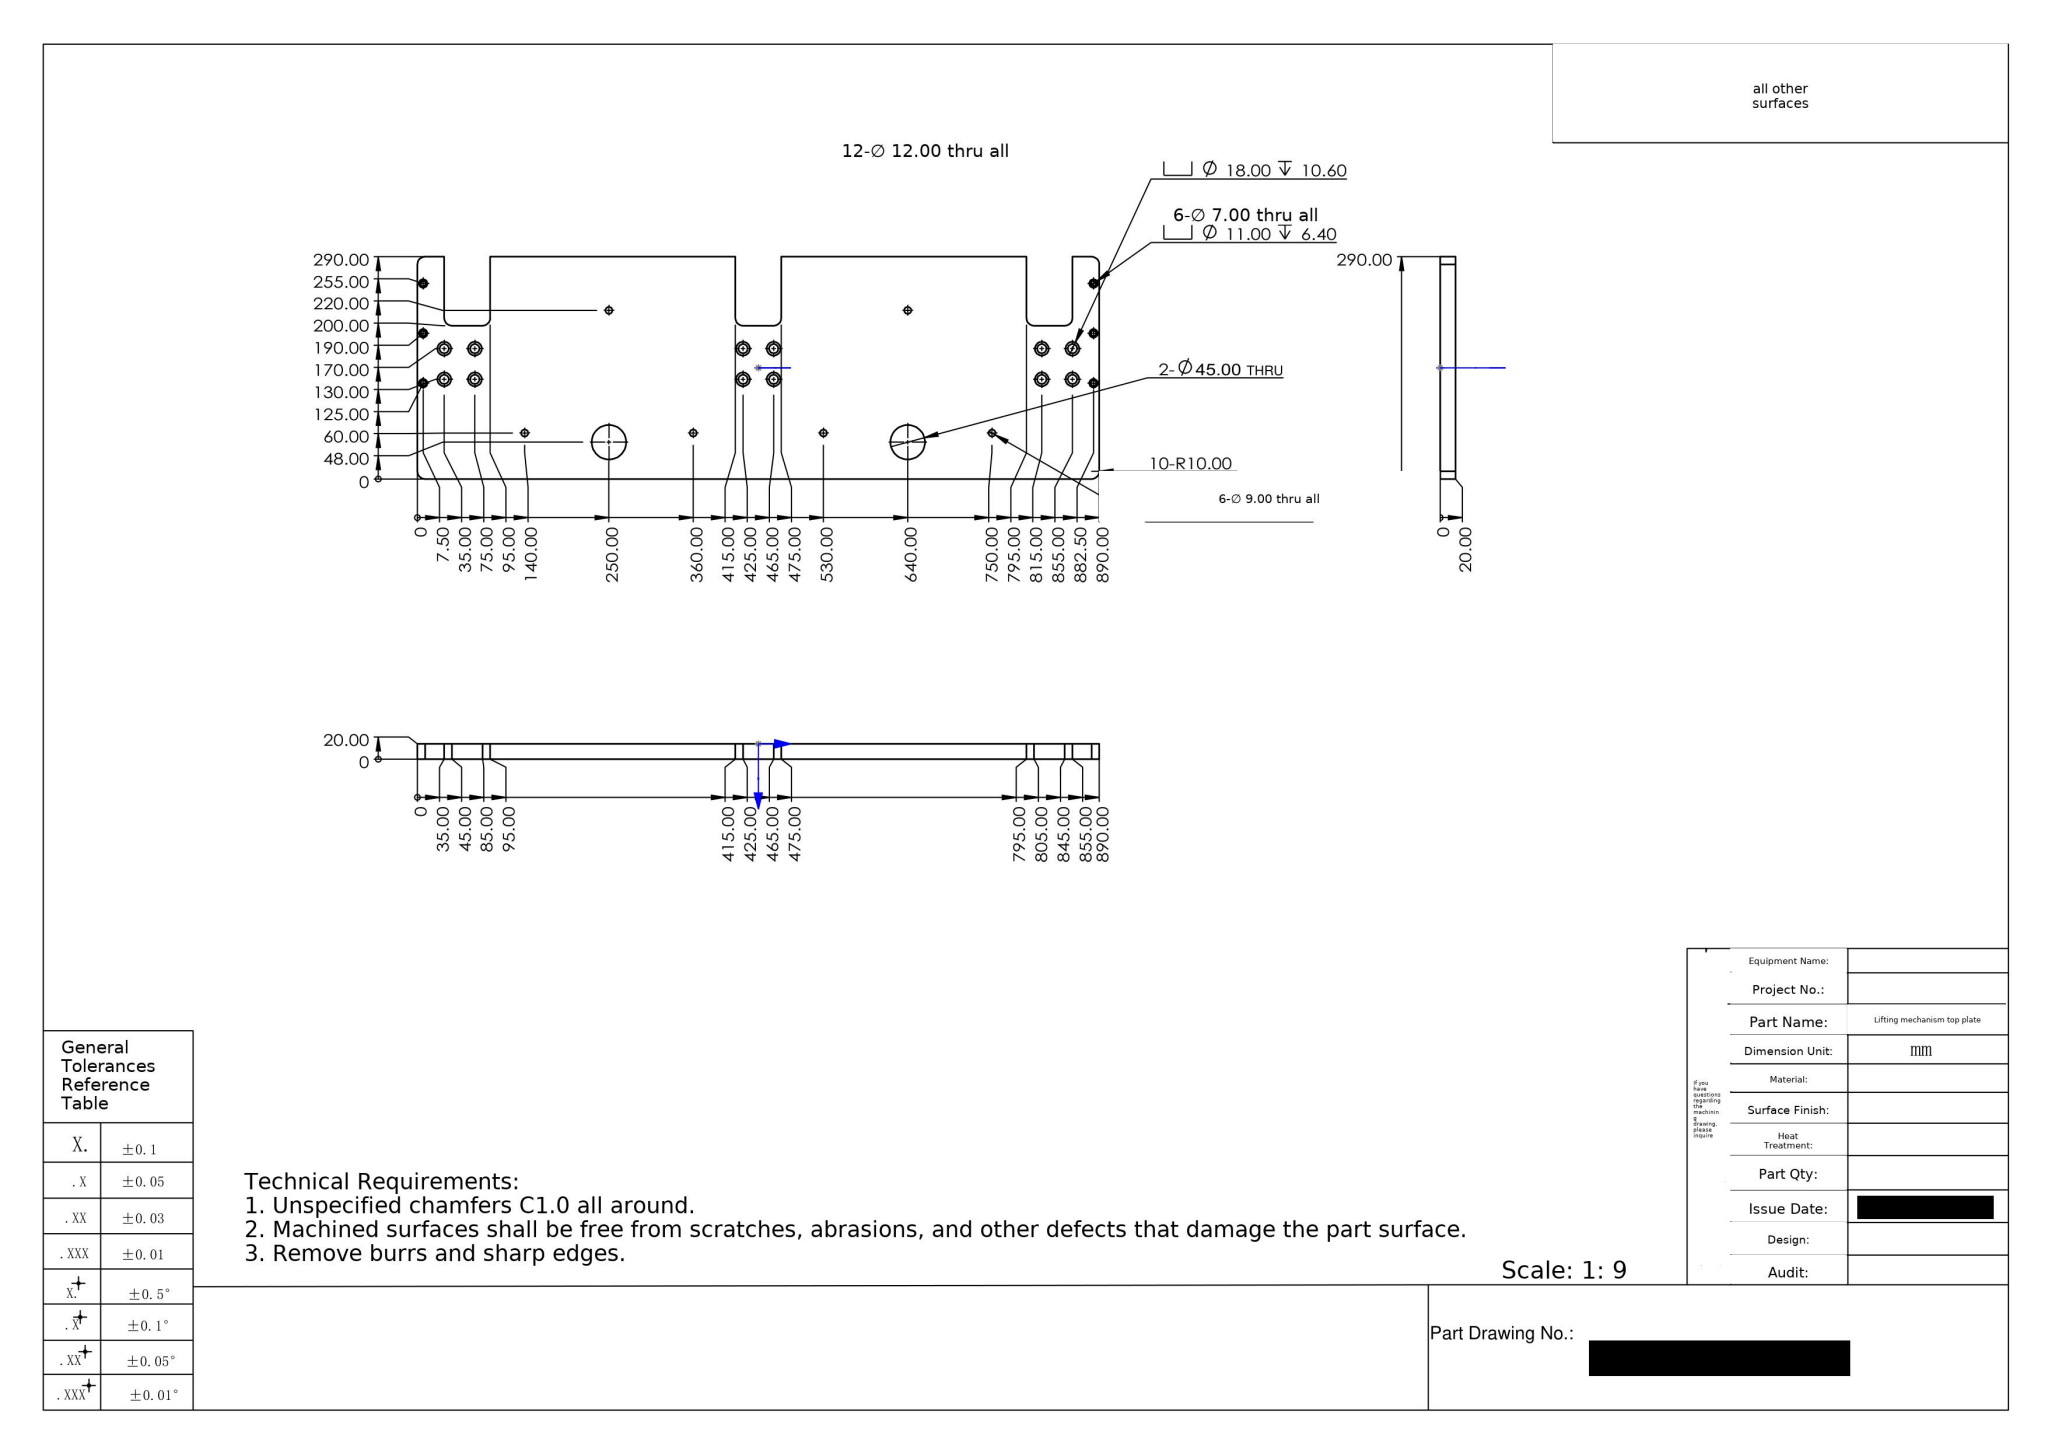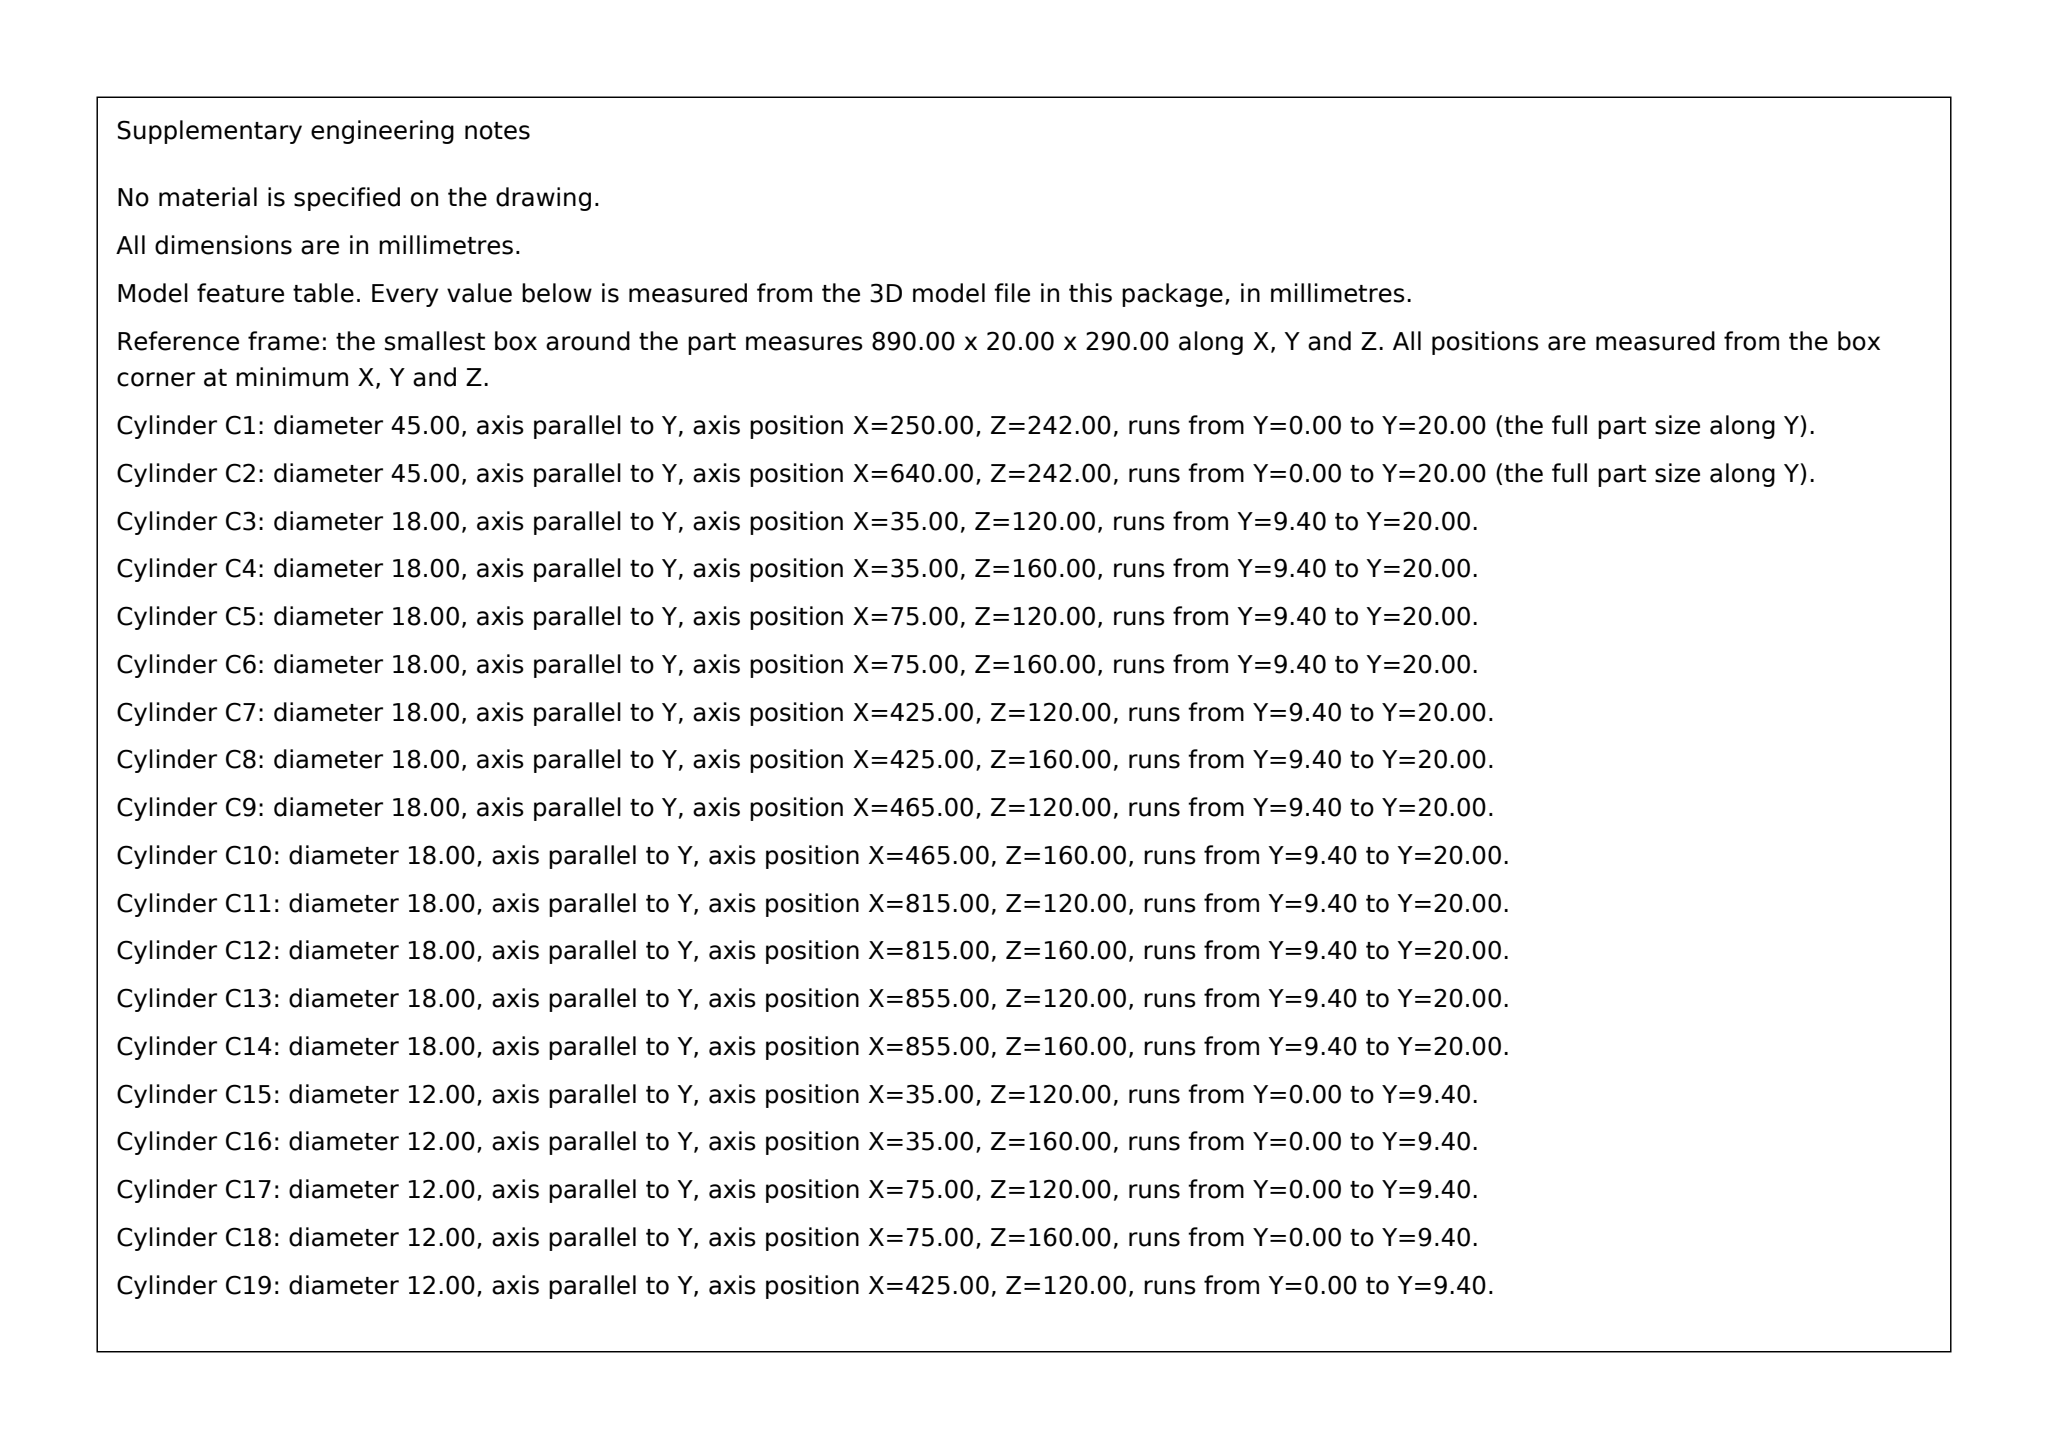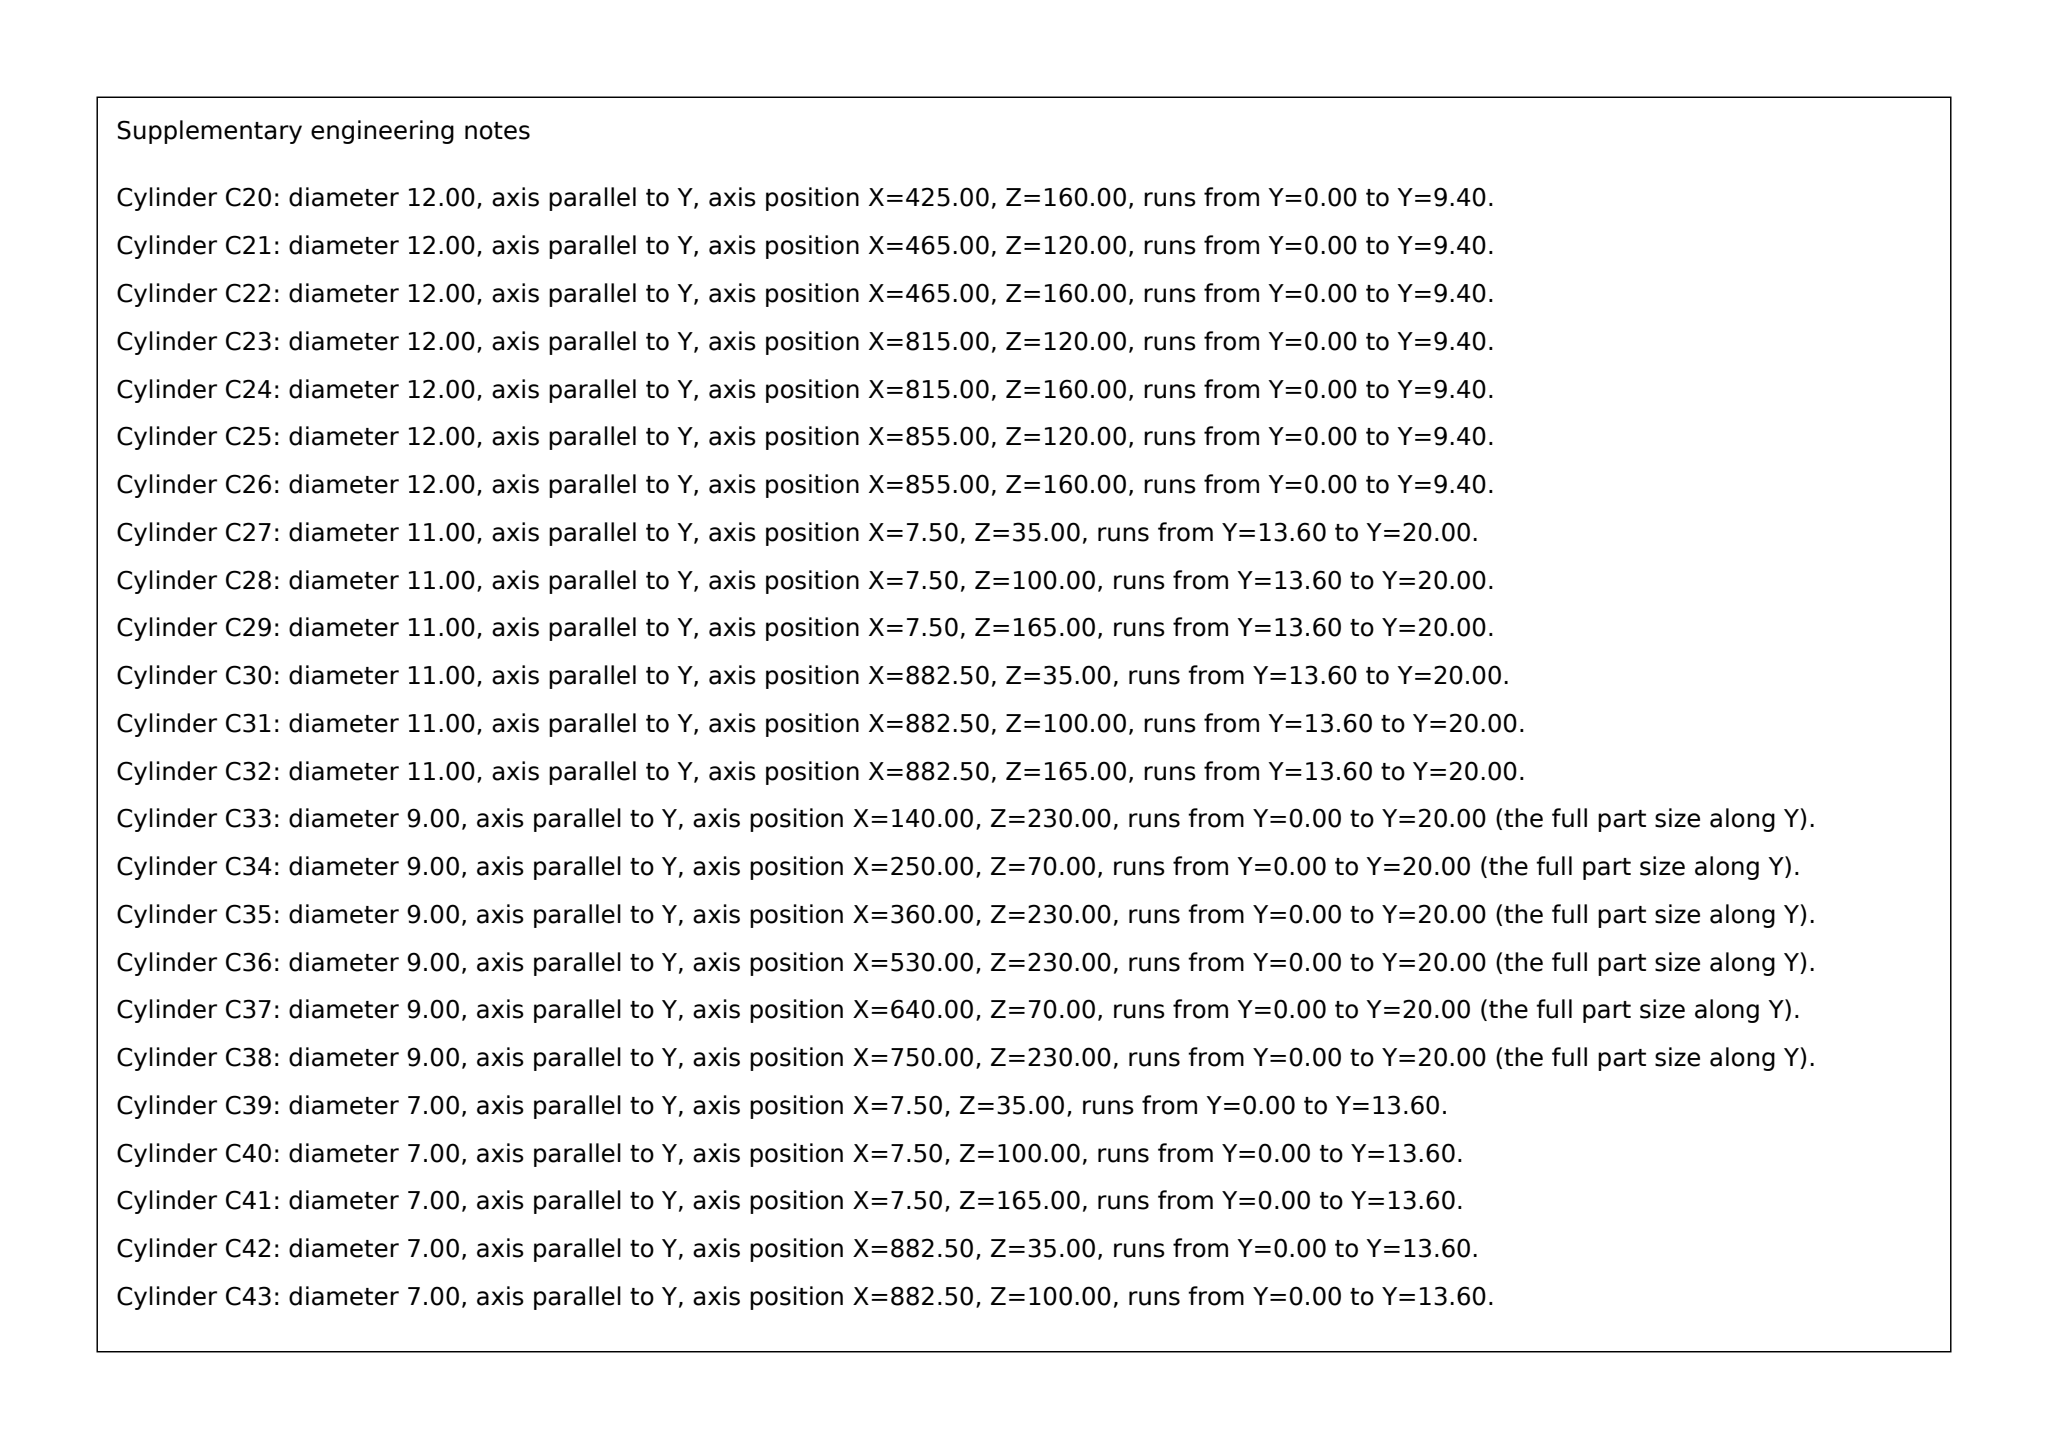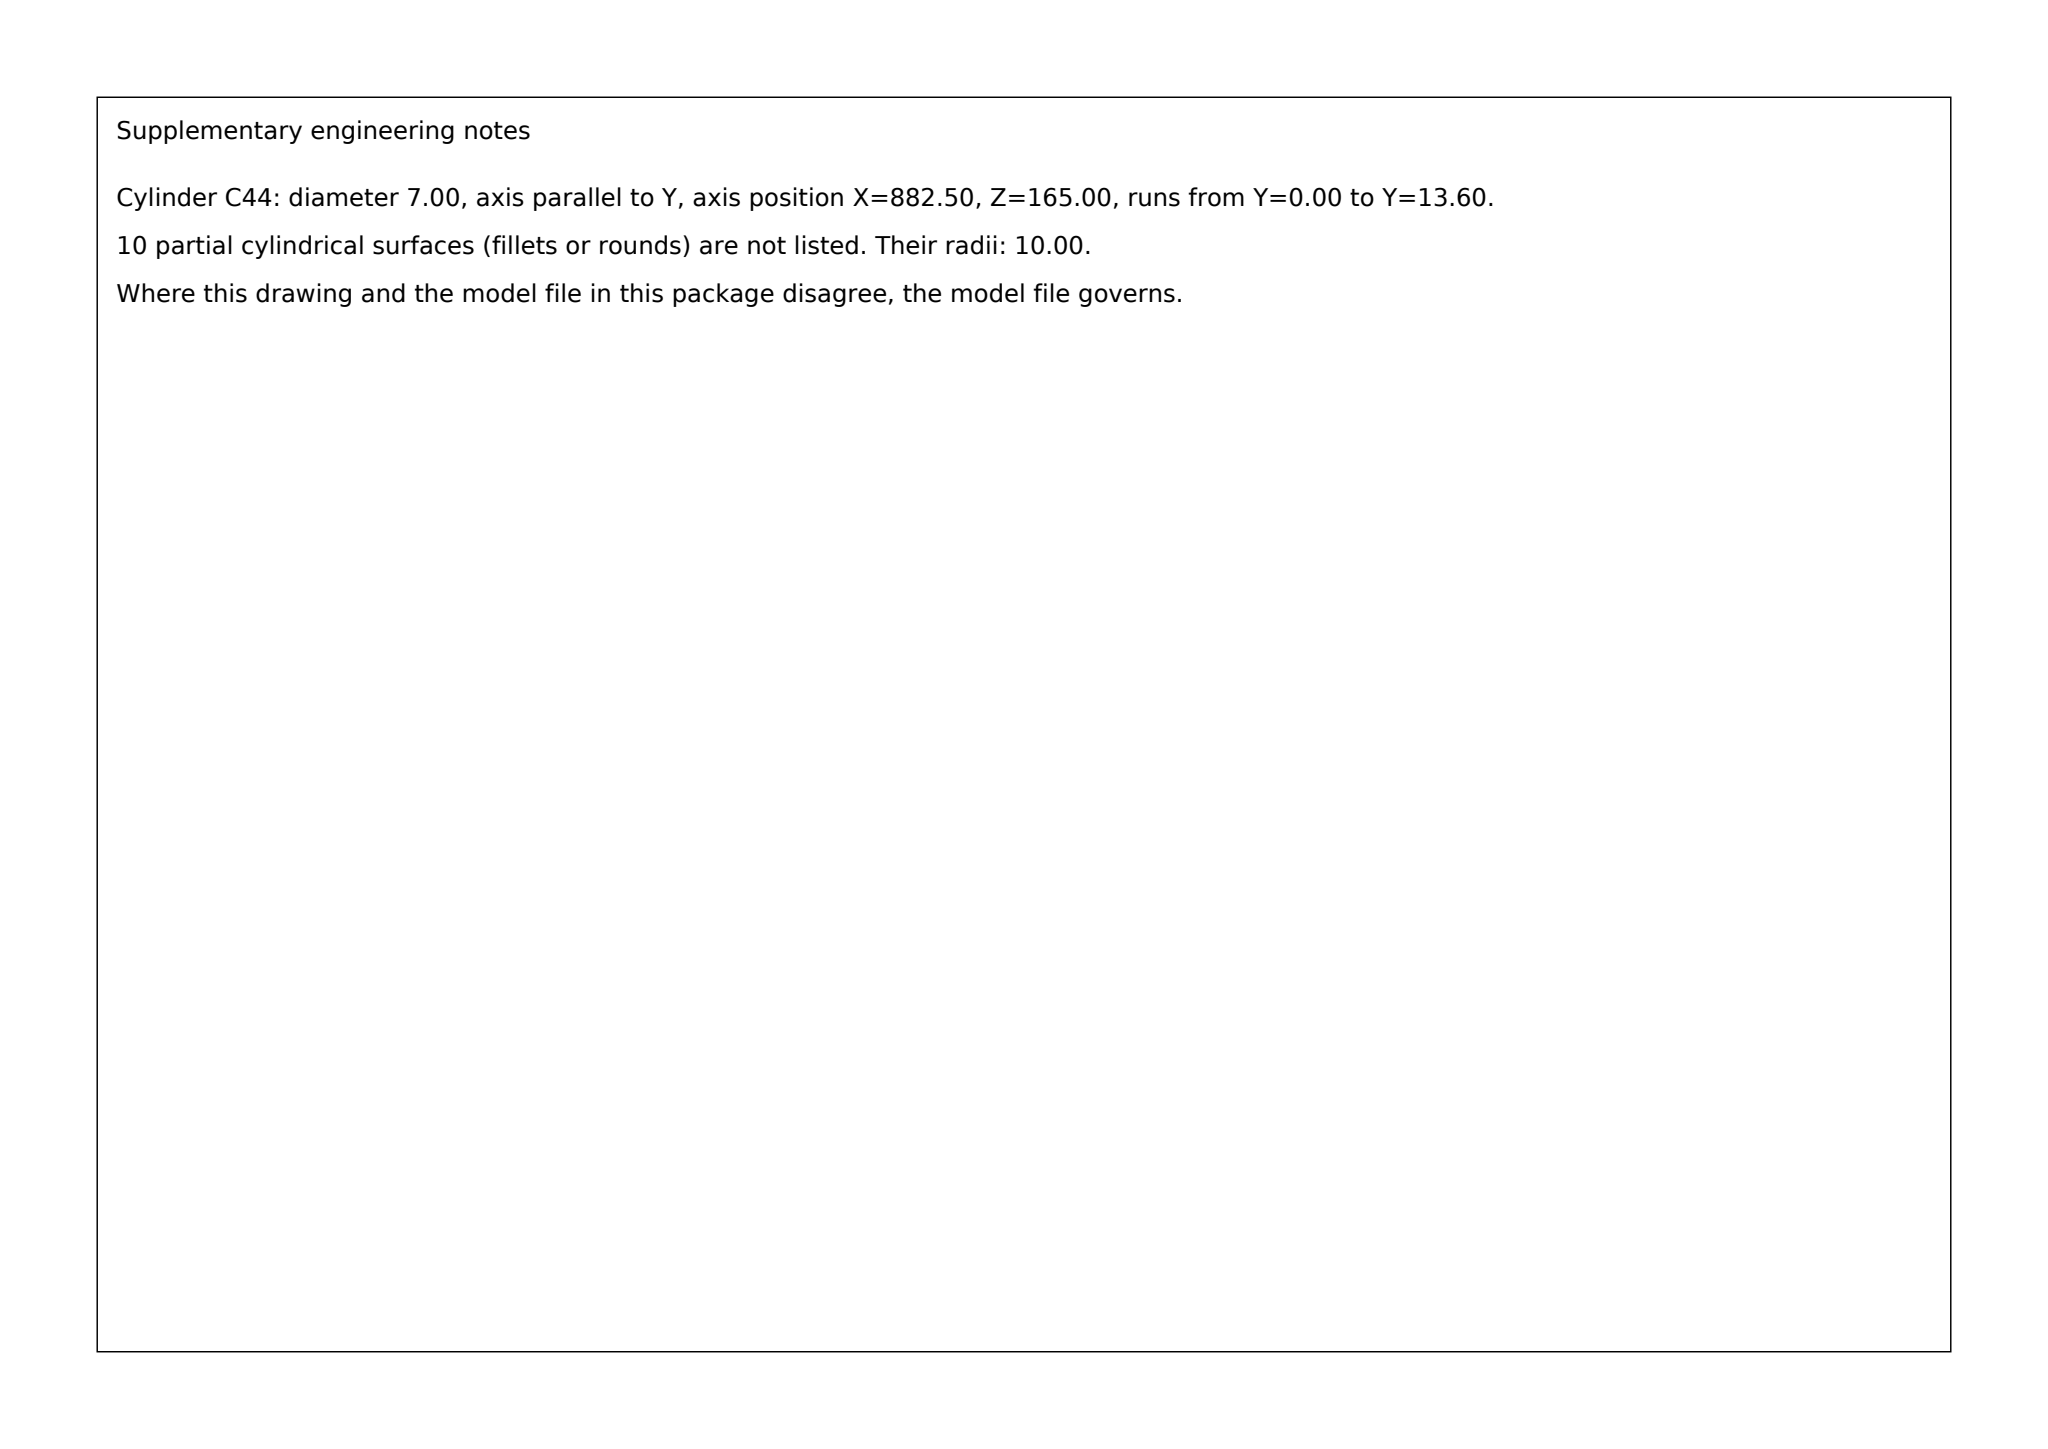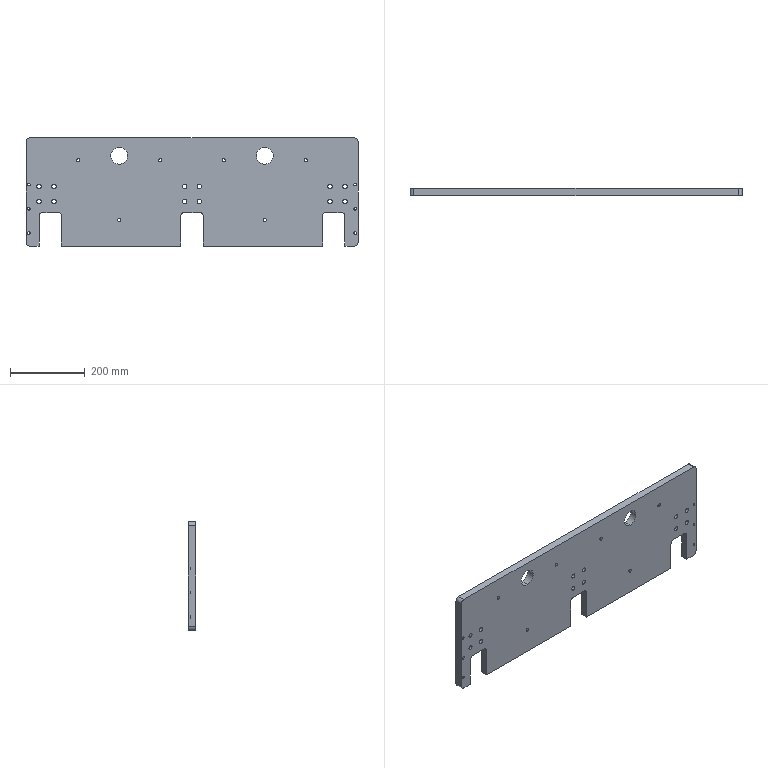Part | SolidWorks | mm | 1 solid | 134 faces | box 890 x 20 x 290 mm | volume 4715692 mm3 | cylinder 98 | plane 36 | commonest cylinder face diameters 18 x24 12 x24 11 x12 7 x12 9 x12 20 x10 45 x4
build123d program:
from build123d import *

# Parameters (mm, degrees)
SKETCH1_W                                        = 890
SKETCH1_H                                        = 290
BOSS_EXTRUDE1_DEPTH                              = 20
M8_CLEARANCE_HOLE2_D                             = 9
CUT_EXTRUDE1_DEPTH                               = 469.455
FILLET2_R                                        = 10
SKETCH15_R                                       = 22.5
CUT_EXTRUDE2_DEPTH                               = 469.455
M6_HEX_SOCKET_HEAD_CAP_SCREW_CBORE1_D            = 7
M6_HEX_SOCKET_HEAD_CAP_SCREW_CBORE1_CBORE_D      = 11
M6_HEX_SOCKET_HEAD_CAP_SCREW_CBORE1_CBORE_DEPTH  = 6.4
M10_HEX_SOCKET_HEAD_CAP_SCREW_CBORE1_D           = 12
M10_HEX_SOCKET_HEAD_CAP_SCREW_CBORE1_CBORE_D     = 18
M10_HEX_SOCKET_HEAD_CAP_SCREW_CBORE1_CBORE_DEPTH = 10.6


with BuildPart() as part:
    # Sketch1 → Boss-Extrude1 (new body)
    with BuildSketch(Plane(origin=(0, 0, 0), x_dir=(1, 0, 0), z_dir=(0, 1, 0))):
        Rectangle(SKETCH1_W, SKETCH1_H)
    extrude(amount=BOSS_EXTRUDE1_DEPTH)

    # M8 Clearance Hole2 (through all)
    with Locations(Plane(origin=(0, 20, 0), x_dir=(1, 0, 0), z_dir=(0, 1, 0))):
        with Locations((195, 75), (-195, 75), (-305, -85), (-85, -85), (85, -85), (305, -85)):
            Hole(M8_CLEARANCE_HOLE2_D / 2)

    # Sketch14 → Cut-Extrude1 (cut, through all)
    with BuildSketch(Plane(origin=(0, 20, 0), x_dir=(1, 0, 0), z_dir=(0, 1, 0))):
        with BuildLine():
            Line((-30, 145), (30, 145))
            Line((30, 145), (30, 65))
            ThreePointArc((30, 65), (27.071, 57.929), (20, 55))
            Line((20, 55), (-20, 55))
            ThreePointArc((-20, 55), (-27.071, 57.929), (-30, 65))
            Line((-30, 65), (-30, 145))
        make_face()
        with BuildLine():
            Line((-410, 145), (-350, 145))
            Line((-350, 145), (-350, 65))
            ThreePointArc((-350, 65), (-352.929, 57.929), (-360, 55))
            Line((-360, 55), (-400, 55))
            ThreePointArc((-400, 55), (-407.071, 57.929), (-410, 65))
            Line((-410, 65), (-410, 145))
        make_face()
        with BuildLine():
            Line((350, 145), (410, 145))
            Line((410, 145), (410, 65))
            ThreePointArc((410, 65), (407.071, 57.929), (400, 55))
            Line((400, 55), (360, 55))
            ThreePointArc((360, 55), (352.929, 57.929), (350, 65))
            Line((350, 65), (350, 145))
        make_face()
    extrude(amount=-CUT_EXTRUDE1_DEPTH, mode=Mode.SUBTRACT)

    # Fillet2
    fillet2_edges = [part.edges().sort_by_distance(p)[0] for p in [
        (-445, 10, -145),
        (445, 10, -145),
        (445, 10, 145),
        (-445, 10, 145),
    ]]
    fillet(fillet2_edges, radius=FILLET2_R)

    # Sketch15 → Cut-Extrude2 (cut, through all)
    with BuildSketch(Plane(origin=(0, 20, 0), x_dir=(1, 0, 0), z_dir=(0, 1, 0))):
        with Locations(Location((-195, -97, 0), (0, 0, 270))):
            Circle(SKETCH15_R)
        with Locations(Location((195, -97, 0), (0, 0, 270))):
            Circle(SKETCH15_R)
    extrude(amount=-CUT_EXTRUDE2_DEPTH, mode=Mode.SUBTRACT)

    # M6 Hex Socket Head Cap Screw CBORE1 (through all)
    with Locations(Plane(origin=(0, 20, 0), x_dir=(1, 0, 0), z_dir=(0, 1, 0))):
        with Locations((437.5, -20), (437.5, 45), (437.5, 110), (-437.5, -20), (-437.5, 45), (-437.5, 110)):
            CounterBoreHole(M6_HEX_SOCKET_HEAD_CAP_SCREW_CBORE1_D / 2, M6_HEX_SOCKET_HEAD_CAP_SCREW_CBORE1_CBORE_D / 2, M6_HEX_SOCKET_HEAD_CAP_SCREW_CBORE1_CBORE_DEPTH)

    # M10 Hex Socket Head Cap Screw CBORE1 (through all)
    with Locations(Plane(origin=(0, 20, 0), x_dir=(1, 0, 0), z_dir=(0, 1, 0))):
        with Locations((-410, 25), (-370, 25), (-370, -15), (-410, -15), (-20, 25), (20, 25), (20, -15), (-20, -15), (370, 25), (410, 25), (410, -15), (370, -15)):
            CounterBoreHole(M10_HEX_SOCKET_HEAD_CAP_SCREW_CBORE1_D / 2, M10_HEX_SOCKET_HEAD_CAP_SCREW_CBORE1_CBORE_D / 2, M10_HEX_SOCKET_HEAD_CAP_SCREW_CBORE1_CBORE_DEPTH)


solid = part.part